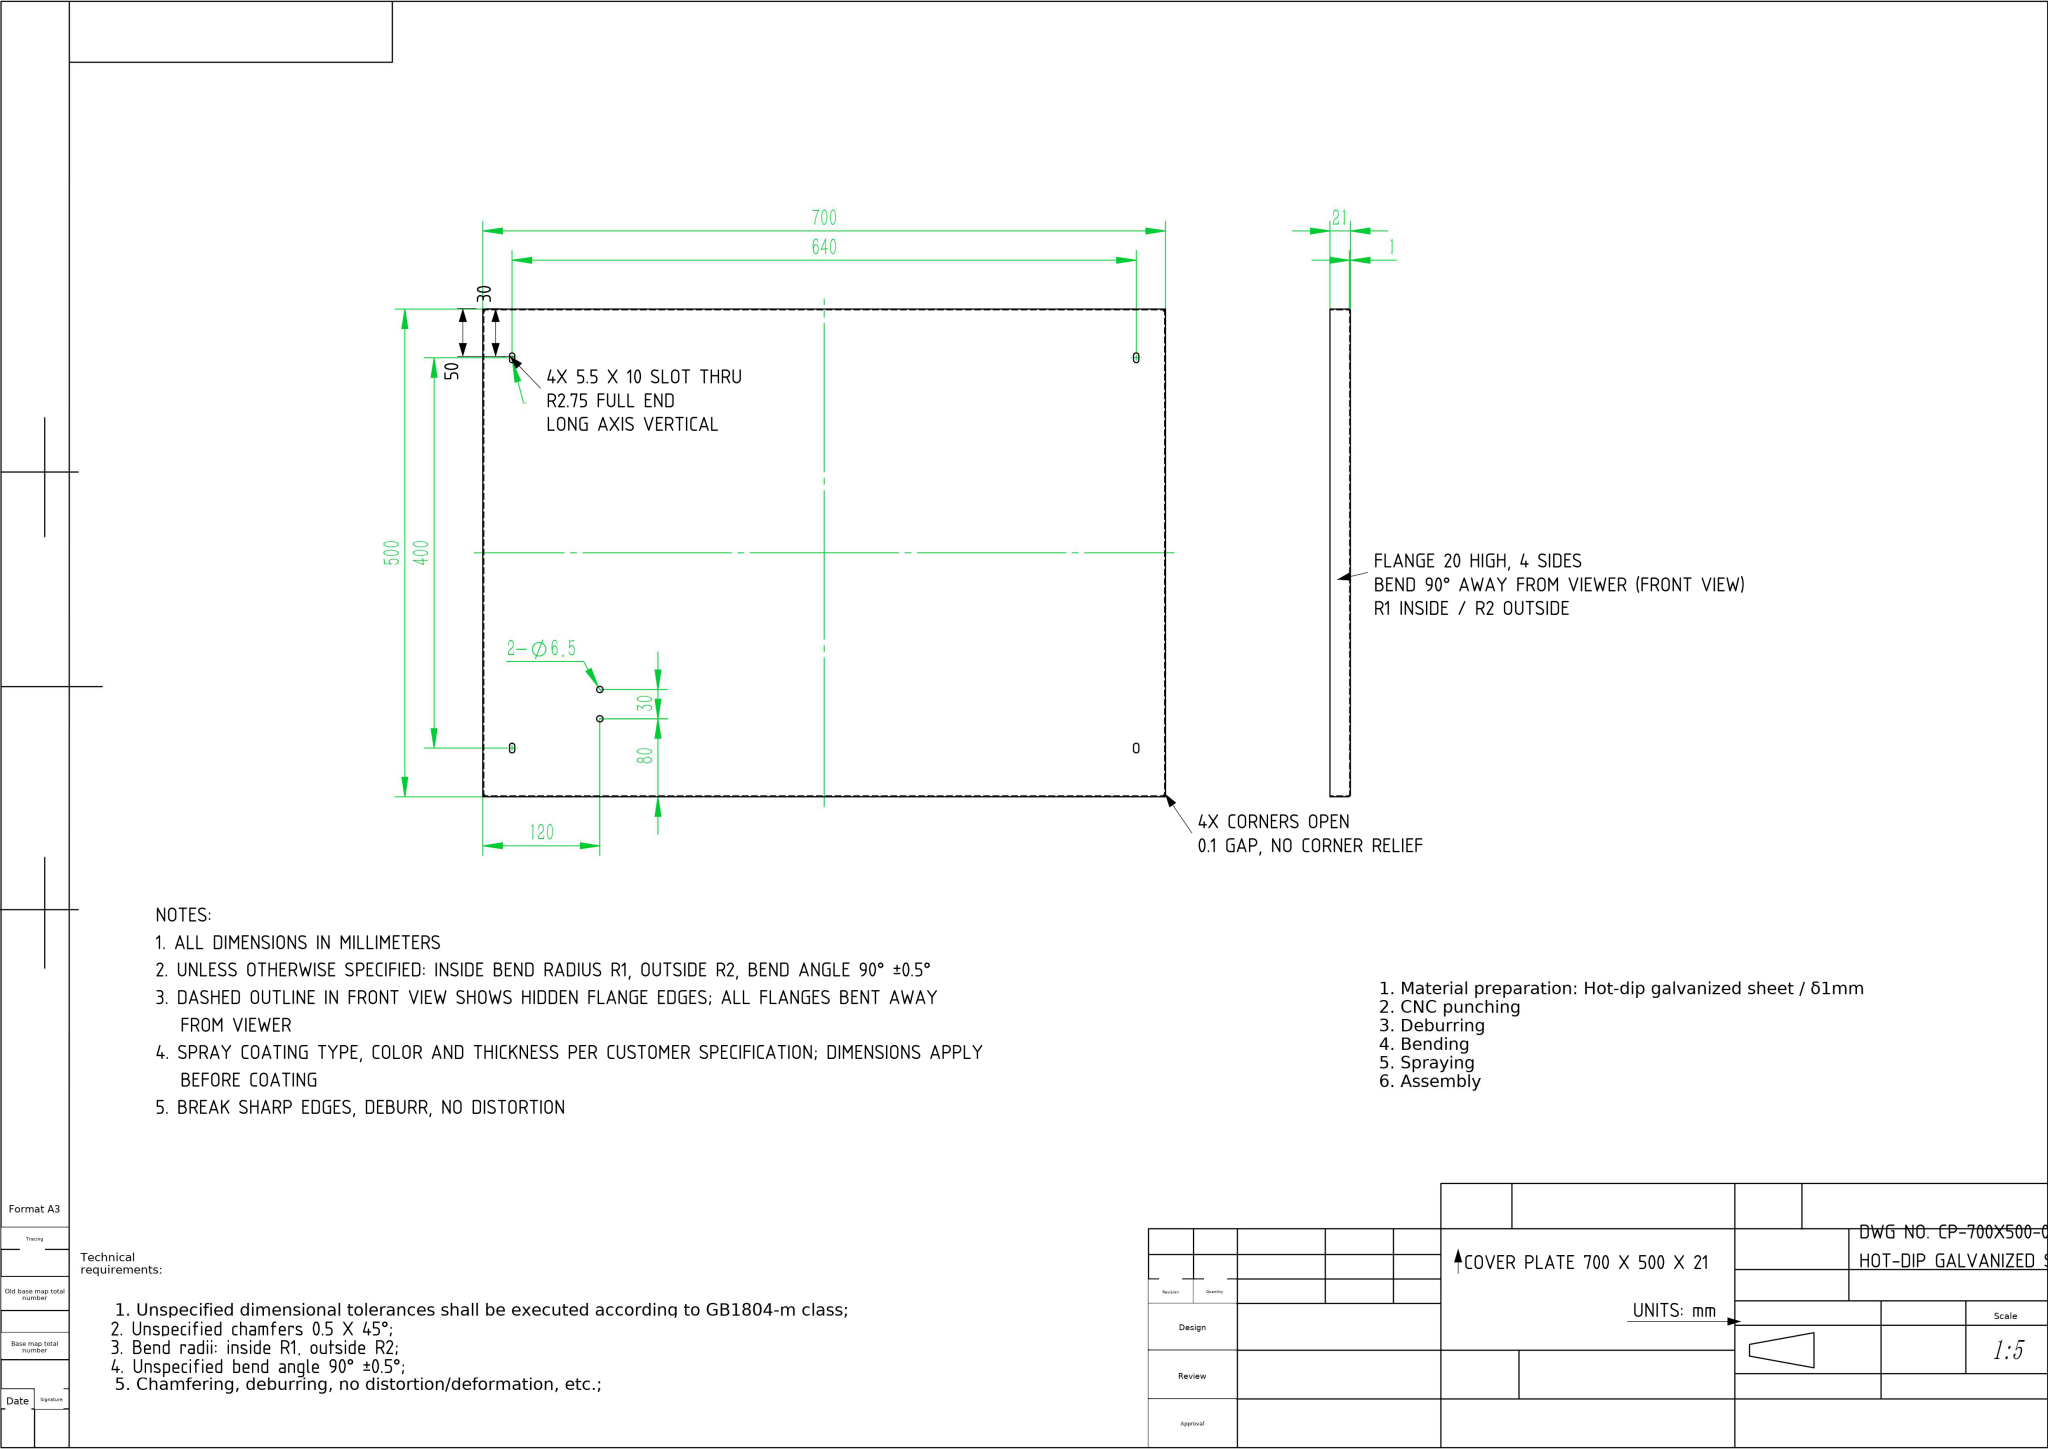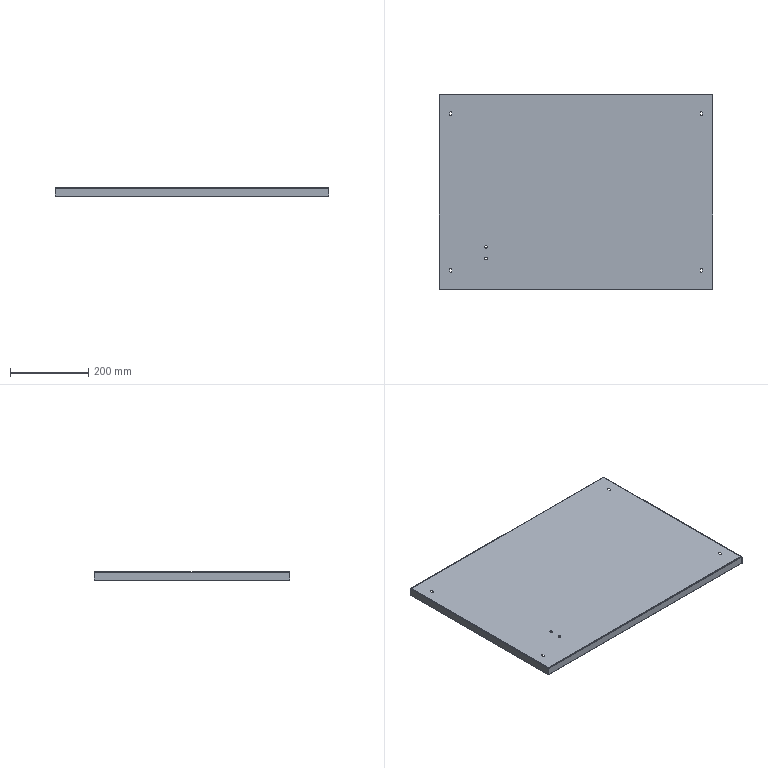Part | NX | mm | 1 solid | 58 faces | box 700 x 500 x 21 mm | volume 396103 mm3 | plane 30 | cylinder 20 | spline 8 | commonest cylinder face diameters 5.5 x8 6.5 x4 2 x4 4 x4